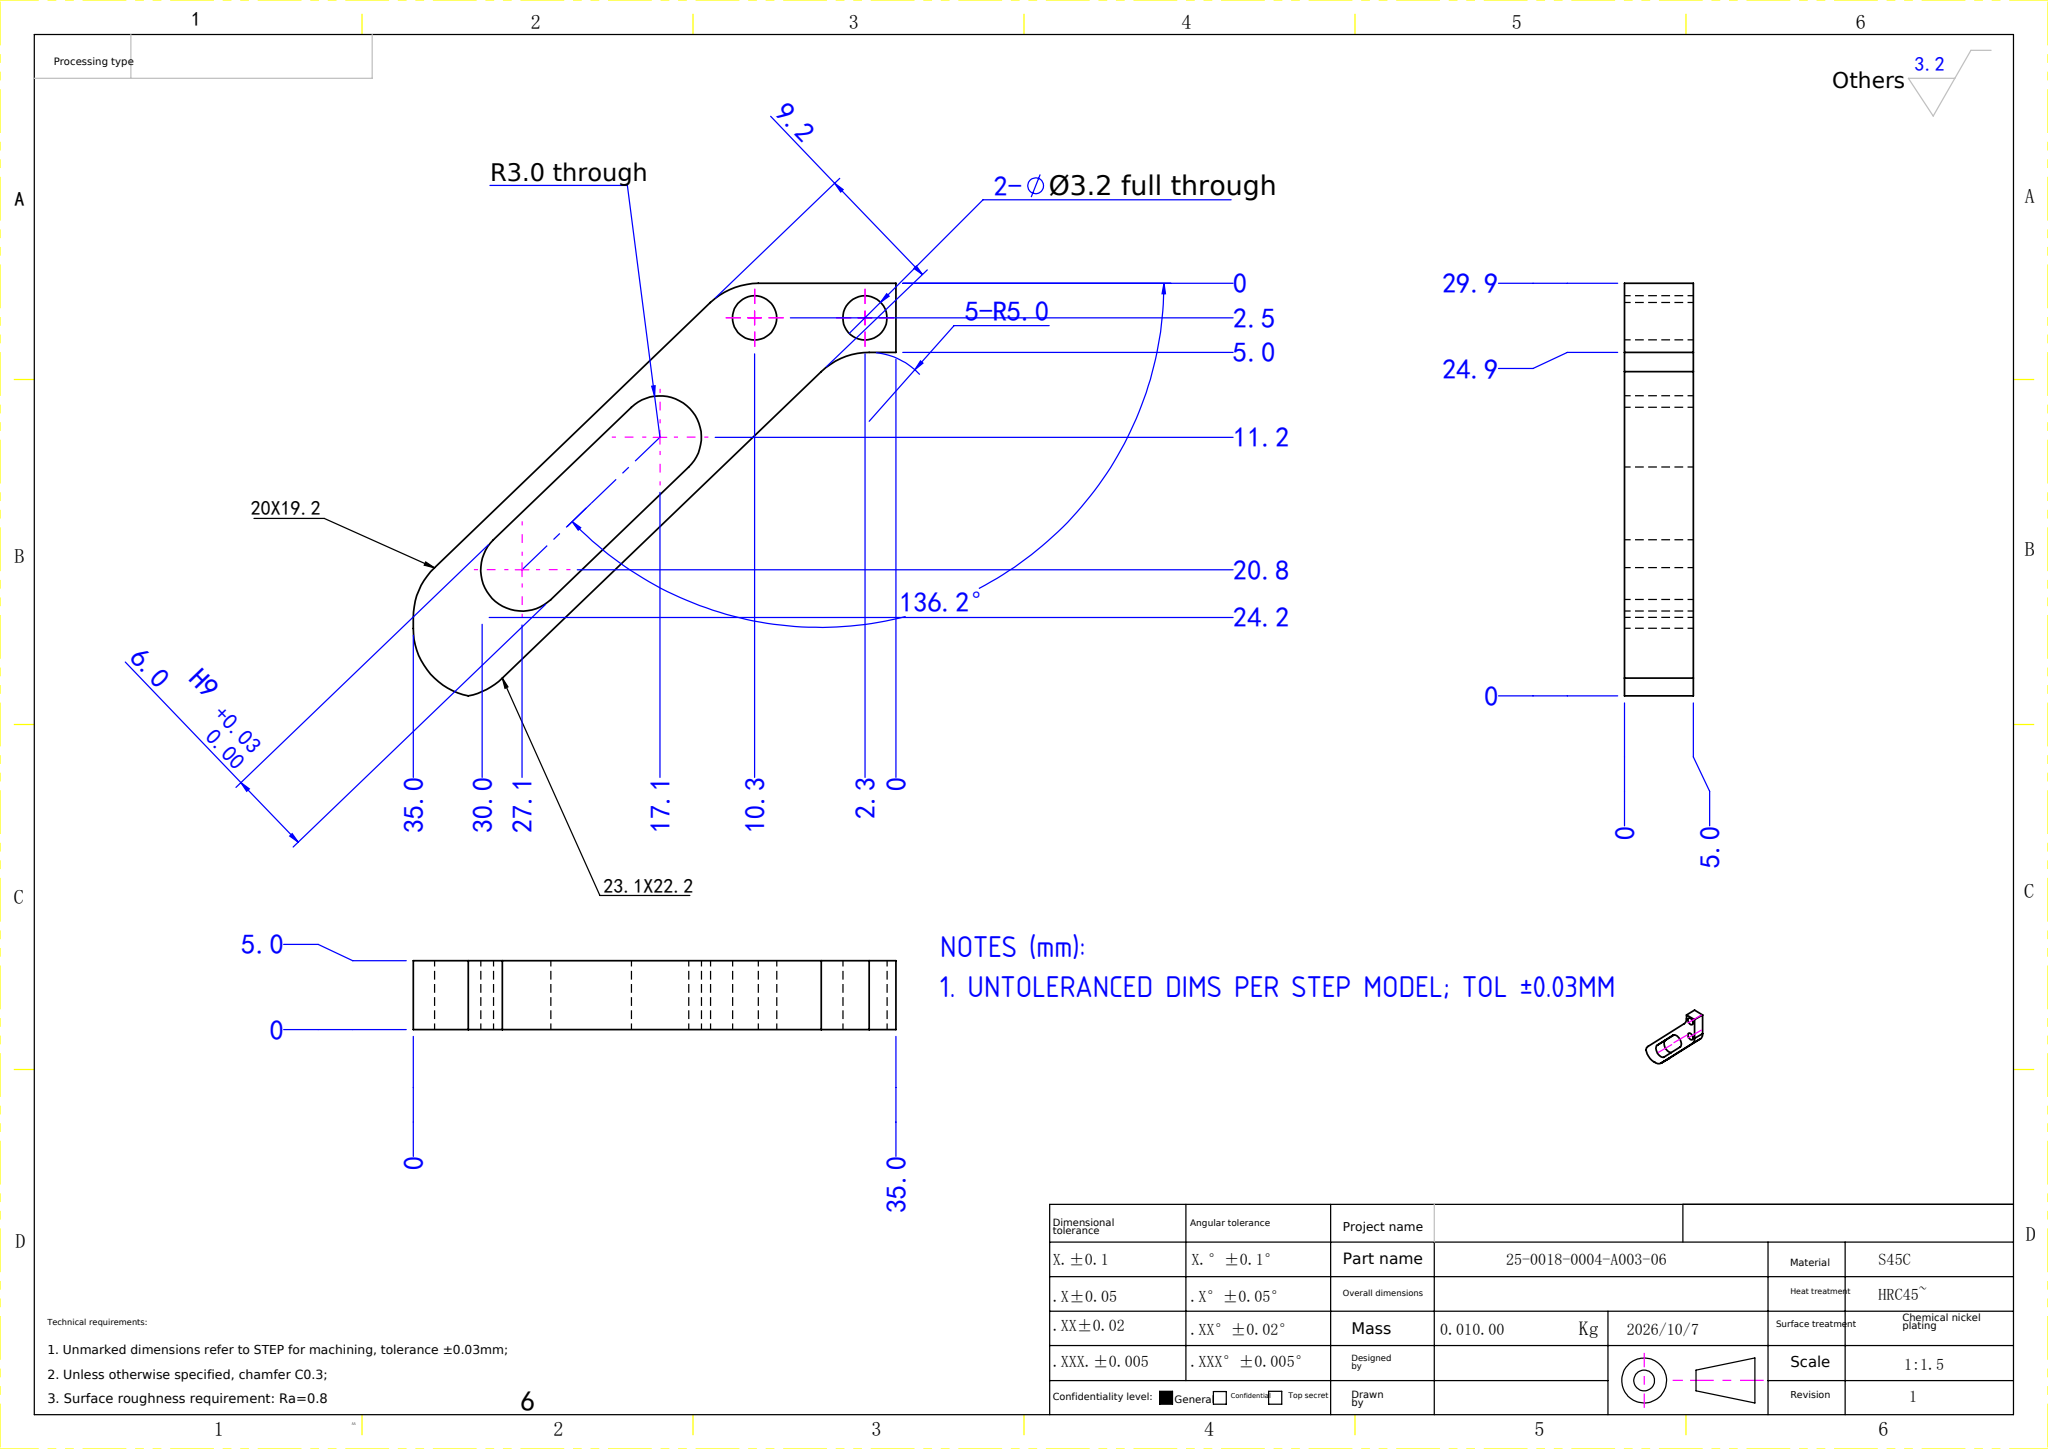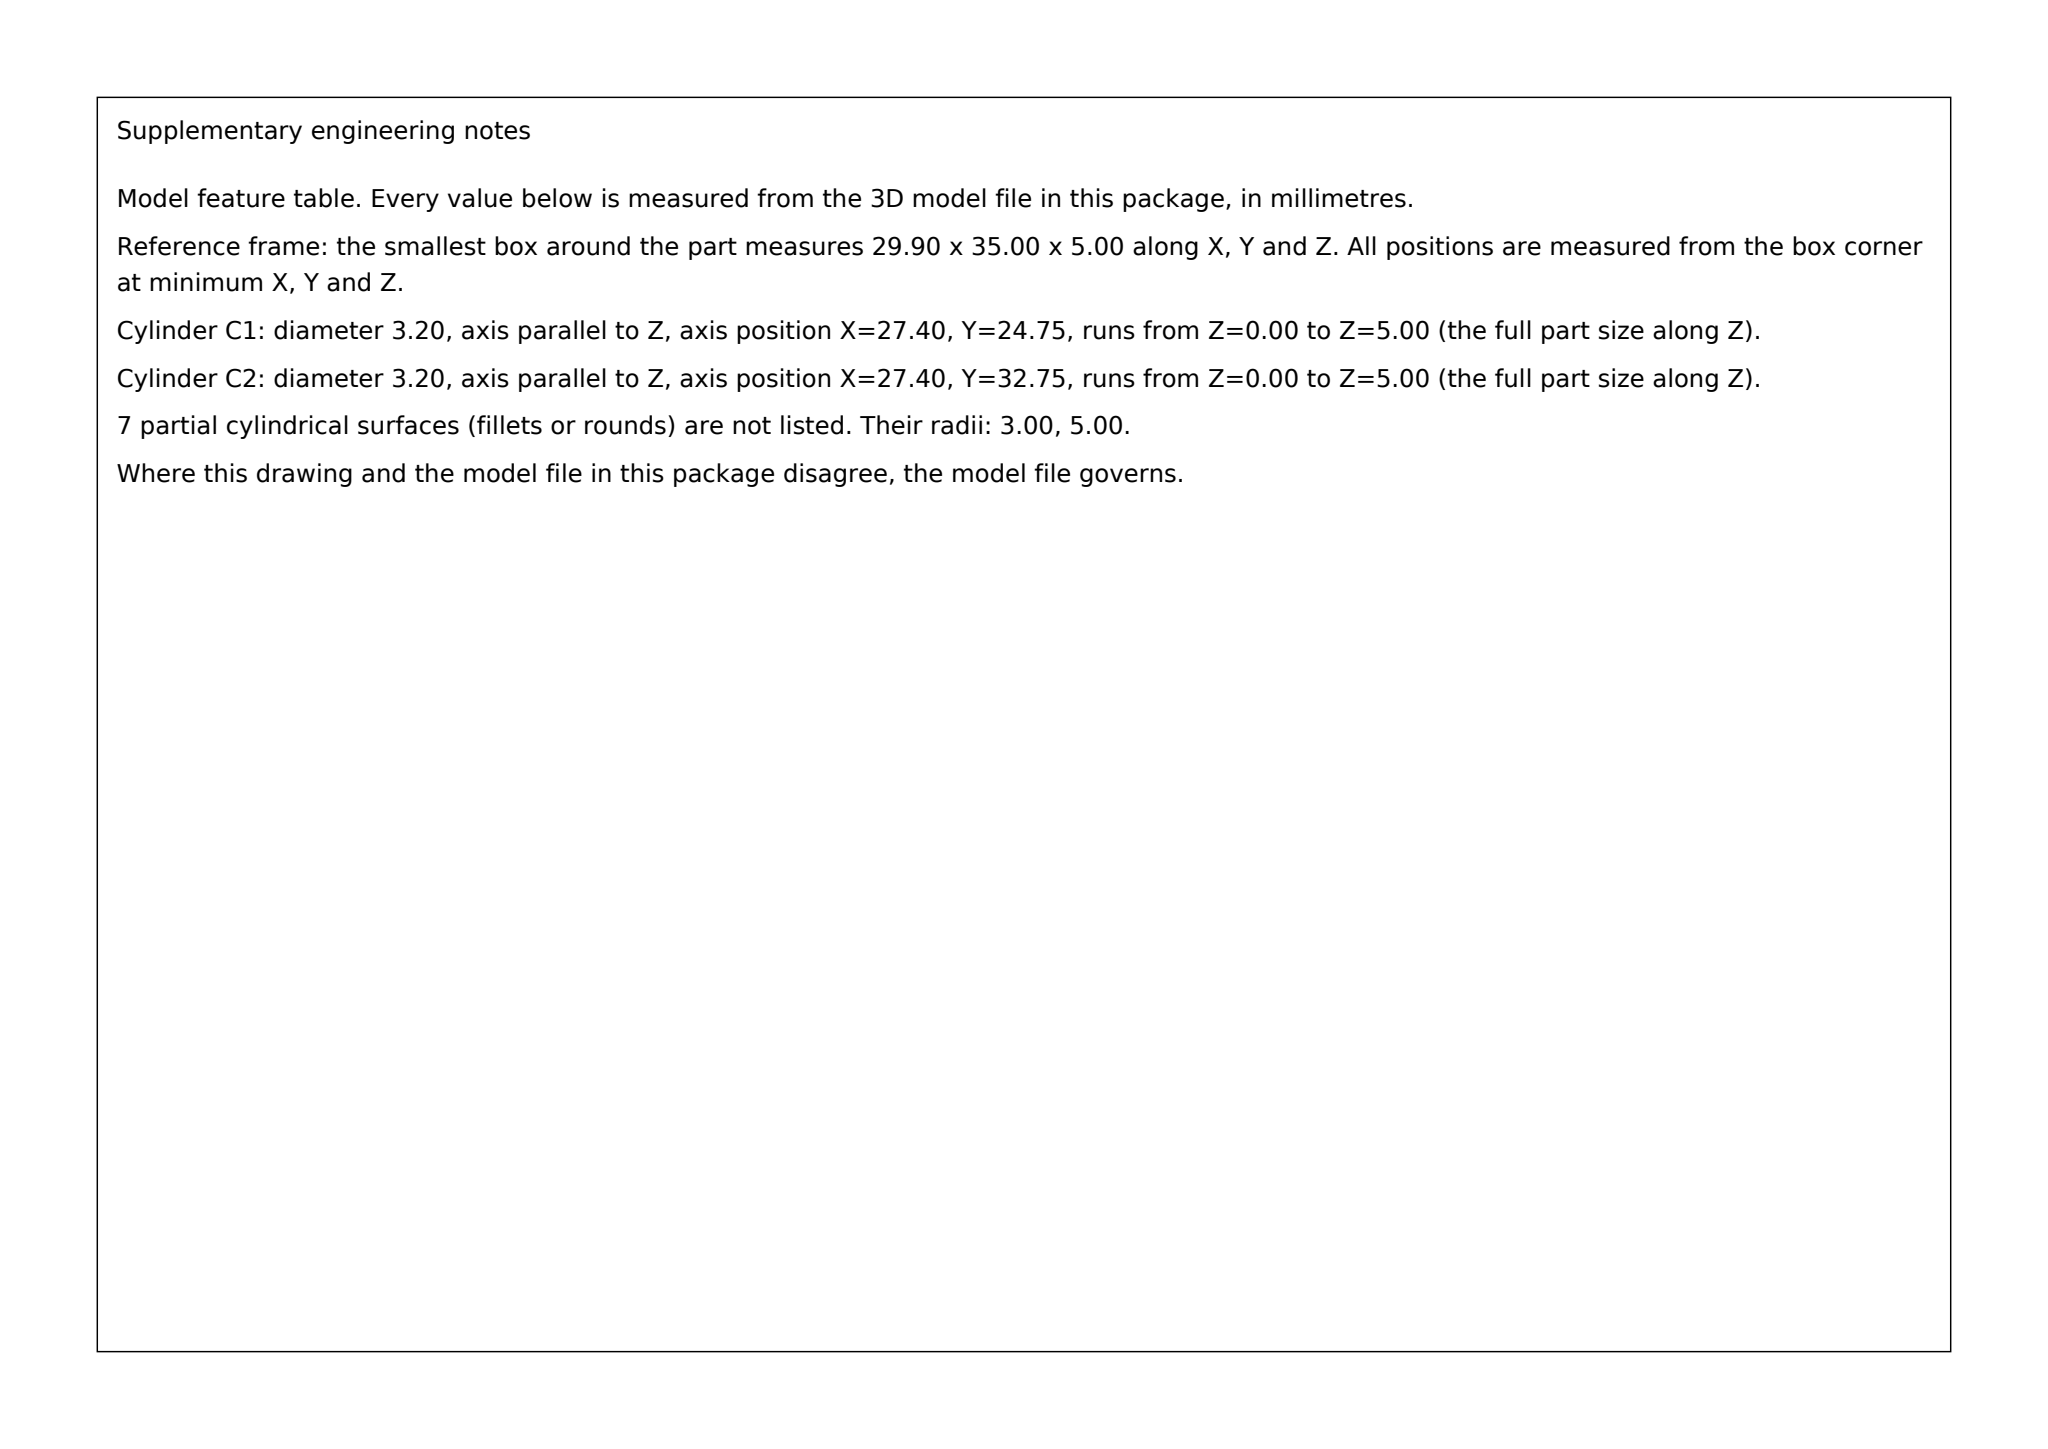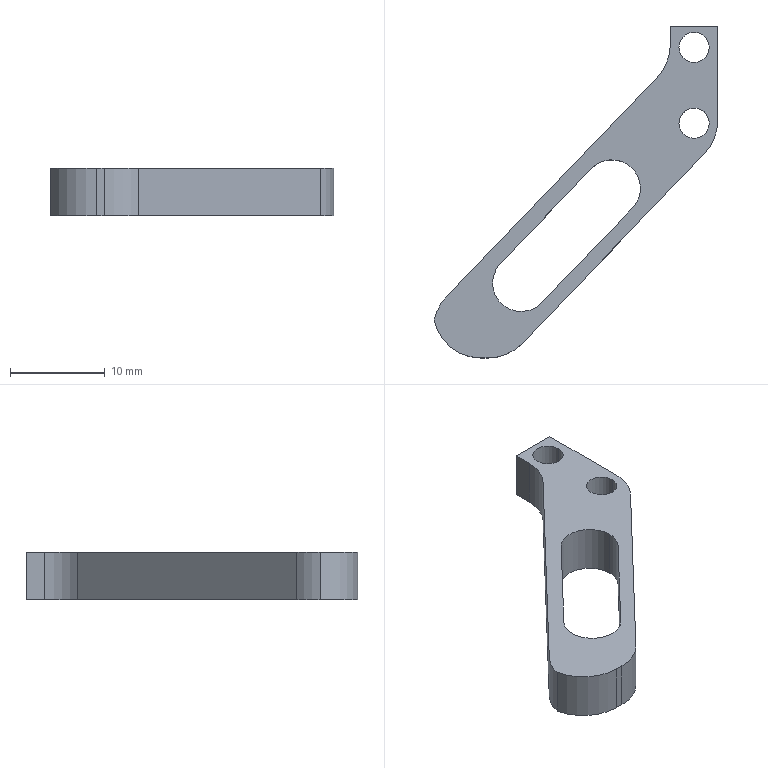Part | SolidWorks | mm | material S45C | 1 solid | 22 faces | box 29.9 x 35 x 5 mm | volume 1188 mm3 | cylinder 12 | plane 10 | commonest cylinder face diameters 10 x5 3.2 x4 6 x3
Drawing notes:
UNTOLERANCED DIMS PER STEP MODEL; TOL ±0.03MM | from the solid: STEP bbox 29.898 x 35.0 x 5.0; all geometry defined in STEP model
STEP:
#1=CARTESIAN_POINT('',(10.9,7.25,-2.5));
#2=VERTEX_POINT('',#1);
#3=CARTESIAN_POINT('',(14.1,7.25,-2.5));
#4=VERTEX_POINT('',#3);
#5=CARTESIAN_POINT('',(12.5,7.25,-2.5));
#6=DIRECTION('',(0.,0.,1.));
#7=DIRECTION('',(1.,0.,0.));
#8=AXIS2_PLACEMENT_3D('',#5,#6,#7);
#9=CIRCLE('',#8,1.6);
#10=EDGE_CURVE('',#2,#4,#9,.T.);
#11=ORIENTED_EDGE('',*,*,#10,.F.);
#12=CARTESIAN_POINT('',(10.9,7.25,2.5));
#13=VERTEX_POINT('',#12);
#14=CARTESIAN_POINT('',(10.9,7.25,2.5));
#15=DIRECTION('',(0.,0.,1.));
#16=VECTOR('',#15,1000.);
#17=LINE('',#14,#16);
#18=EDGE_CURVE('',#2,#13,#17,.T.);
#19=ORIENTED_EDGE('',*,*,#18,.T.);
#20=CARTESIAN_POINT('',(14.1,7.25,2.5));
#21=VERTEX_POINT('',#20);
#22=CARTESIAN_POINT('',(12.5,7.25,2.5));
#23=DIRECTION('',(0.,0.,1.));
#24=DIRECTION('',(1.,0.,0.));
#25=AXIS2_PLACEMENT_3D('',#22,#23,#24);
#26=CIRCLE('',#25,1.6);
#27=EDGE_CURVE('',#13,#21,#26,.T.);
#28=ORIENTED_EDGE('',*,*,#27,.T.);
#29=CARTESIAN_POINT('',(14.1,7.25,2.5));
#30=DIRECTION('',(0.,0.,1.));
#31=VECTOR('',#30,1000.);
#32=LINE('',#29,#31);
#33=EDGE_CURVE('',#4,#21,#32,.T.);
#34=ORIENTED_EDGE('',*,*,#33,.F.);
#35=EDGE_LOOP('',(#11,#19,#28,#34));
#36=FACE_OUTER_BOUND('',#35,.T.);
#37=CARTESIAN_POINT('',(12.5,7.25,2.5));
#38=DIRECTION('',(0.,0.,1.));
#39=DIRECTION('',(1.,0.,0.));
#40=AXIS2_PLACEMENT_3D('',#37,#38,#39);
#41=CYLINDRICAL_SURFACE('',#40,1.6);
#42=ADVANCED_FACE('',(#36),#41,.F.);
#43=CARTESIAN_POINT('',(10.9,15.25,-2.5));
#44=VERTEX_POINT('',#43);
#45=CARTESIAN_POINT('',(14.1,15.25,-2.5));
#46=VERTEX_POINT('',#45);
#47=CARTESIAN_POINT('',(12.5,15.25,-2.5));
#48=DIRECTION('',(0.,0.,1.));
#49=DIRECTION('',(1.,0.,0.));
#50=AXIS2_PLACEMENT_3D('',#47,#48,#49);
#51=CIRCLE('',#50,1.6);
#52=EDGE_CURVE('',#44,#46,#51,.T.);
#53=ORIENTED_EDGE('',*,*,#52,.F.);
#54=CARTESIAN_POINT('',(10.9,15.25,2.5));
#55=VERTEX_POINT('',#54);
#56=CARTESIAN_POINT('',(10.9,15.25,2.5));
#57=DIRECTION('',(0.,0.,1.));
#58=VECTOR('',#57,1000.);
#59=LINE('',#56,#58);
#60=EDGE_CURVE('',#44,#55,#59,.T.);
#61=ORIENTED_EDGE('',*,*,#60,.T.);
#62=CARTESIAN_POINT('',(14.1,15.25,2.5));
#63=VERTEX_POINT('',#62);
#64=CARTESIAN_POINT('',(12.5,15.25,2.5));
#65=DIRECTION('',(0.,0.,1.));
#66=DIRECTION('',(1.,0.,0.));
#67=AXIS2_PLACEMENT_3D('',#64,#65,#66);
#68=CIRCLE('',#67,1.6);
#69=EDGE_CURVE('',#55,#63,#68,.T.);
#70=ORIENTED_EDGE('',*,*,#69,.T.);
#71=CARTESIAN_POINT('',(14.1,15.25,2.5));
#72=DIRECTION('',(0.,0.,1.));
#73=VECTOR('',#72,1000.);
#74=LINE('',#71,#73);
#75=EDGE_CURVE('',#46,#63,#74,.T.);
#76=ORIENTED_EDGE('',*,*,#75,.F.);
#77=EDGE_LOOP('',(#53,#61,#70,#76));
#78=FACE_OUTER_BOUND('',#77,.T.);
#79=CARTESIAN_POINT('',(12.5,15.25,2.5));
#80=DIRECTION('',(0.,0.,1.));
#81=DIRECTION('',(1.,0.,0.));
#82=AXIS2_PLACEMENT_3D('',#79,#80,#81);
#83=CYLINDRICAL_SURFACE('',#82,1.6);
#84=ADVANCED_FACE('',(#78),#83,.F.);
#85=CARTESIAN_POINT('',(6.85,0.39,-2.5));
#86=VERTEX_POINT('',#85);
#87=CARTESIAN_POINT('',(1.686,2.468,-2.5));
#88=VERTEX_POINT('',#87);
#89=CARTESIAN_POINT('',(3.85,0.39,-2.5));
#90=DIRECTION('',(0.,0.,1.));
#91=DIRECTION('',(1.,0.,0.));
#92=AXIS2_PLACEMENT_3D('',#89,#90,#91);
#93=CIRCLE('',#92,3.);
#94=EDGE_CURVE('',#86,#88,#93,.T.);
#95=ORIENTED_EDGE('',*,*,#94,.F.);
#96=CARTESIAN_POINT('',(6.85,0.39,2.5));
#97=VERTEX_POINT('',#96);
#98=CARTESIAN_POINT('',(6.85,0.39,-2.5));
#99=DIRECTION('',(0.,0.,1.));
#100=VECTOR('',#99,1000.);
#101=LINE('',#98,#100);
#102=EDGE_CURVE('',#86,#97,#101,.T.);
#103=ORIENTED_EDGE('',*,*,#102,.T.);
#104=CARTESIAN_POINT('',(1.686,2.468,2.5));
#105=VERTEX_POINT('',#104);
#106=CARTESIAN_POINT('',(3.85,0.39,2.5));
#107=DIRECTION('',(0.,0.,1.));
#108=DIRECTION('',(1.,0.,0.));
#109=AXIS2_PLACEMENT_3D('',#106,#107,#108);
#110=CIRCLE('',#109,3.);
#111=EDGE_CURVE('',#97,#105,#110,.T.);
#112=ORIENTED_EDGE('',*,*,#111,.T.);
#113=CARTESIAN_POINT('',(1.686,2.468,-7.5));
#114=DIRECTION('',(0.,0.,1.));
#115=VECTOR('',#114,1000.);
#116=LINE('',#113,#115);
#117=EDGE_CURVE('',#88,#105,#116,.T.);
#118=ORIENTED_EDGE('',*,*,#117,.F.);
#119=EDGE_LOOP('',(#95,#103,#112,#118));
#120=FACE_OUTER_BOUND('',#119,.T.);
#121=CARTESIAN_POINT('',(3.85,0.39,-2.5));
#122=DIRECTION('',(0.,0.,1.));
#123=DIRECTION('',(1.,0.,0.));
#124=AXIS2_PLACEMENT_3D('',#121,#122,#123);
#125=CYLINDRICAL_SURFACE('',#124,3.);
#126=ADVANCED_FACE('',(#120),#125,.F.);
#127=CARTESIAN_POINT('',(12.5,7.25,2.5));
#128=DIRECTION('',(0.,0.,1.));
#129=DIRECTION('',(1.,0.,0.));
#130=AXIS2_PLACEMENT_3D('',#127,#128,#129);
#131=CIRCLE('',#130,1.6);
#132=EDGE_CURVE('',#21,#13,#131,.T.);
#133=ORIENTED_EDGE('',*,*,#132,.F.);
#134=ORIENTED_EDGE('',*,*,#27,.F.);
#135=EDGE_LOOP('',(#133,#134));
#136=FACE_BOUND('',#135,.T.);
#137=CARTESIAN_POINT('',(6.014,-1.688,2.5));
#138=VERTEX_POINT('',#137);
#139=CARTESIAN_POINT('',(3.85,0.39,2.5));
#140=DIRECTION('',(0.,0.,1.));
#141=DIRECTION('',(1.,0.,0.));
#142=AXIS2_PLACEMENT_3D('',#139,#140,#141);
#143=CIRCLE('',#142,3.);
#144=EDGE_CURVE('',#138,#97,#143,.T.);
#145=ORIENTED_EDGE('',*,*,#144,.F.);
#146=CARTESIAN_POINT('',(-3.586,-11.688,2.5));
#147=VERTEX_POINT('',#146);
#148=CARTESIAN_POINT('',(6.014,-1.688,2.5));
#149=DIRECTION('',(0.6925,0.7214,0.));
#150=VECTOR('',#149,1000.);
#151=LINE('',#148,#150);
#152=EDGE_CURVE('',#147,#138,#151,.T.);
#153=ORIENTED_EDGE('',*,*,#152,.F.);
#154=CARTESIAN_POINT('',(-7.914,-7.532,2.5));
#155=VERTEX_POINT('',#154);
#156=CARTESIAN_POINT('',(-5.75,-9.61,2.5));
#157=DIRECTION('',(0.,0.,1.));
#158=DIRECTION('',(1.,0.,0.));
#159=AXIS2_PLACEMENT_3D('',#156,#157,#158);
#160=CIRCLE('',#159,3.);
#161=EDGE_CURVE('',#155,#147,#160,.T.);
#162=ORIENTED_EDGE('',*,*,#161,.F.);
#163=CARTESIAN_POINT('',(1.686,2.468,2.5));
#164=DIRECTION('',(-0.6925,-0.7214,0.));
#165=VECTOR('',#164,1000.);
#166=LINE('',#163,#165);
#167=EDGE_CURVE('',#105,#155,#166,.T.);
#168=ORIENTED_EDGE('',*,*,#167,.F.);
#169=ORIENTED_EDGE('',*,*,#111,.F.);
#170=EDGE_LOOP('',(#145,#153,#162,#168,#169));
#171=FACE_BOUND('',#170,.T.);
#172=CARTESIAN_POINT('',(-13.607,-11.049,2.5));
#173=VERTEX_POINT('',#172);
#174=CARTESIAN_POINT('',(-14.898,-13.506,2.5));
#175=VERTEX_POINT('',#174);
#176=CARTESIAN_POINT('',(-10.,-14.512,2.5));
#177=DIRECTION('',(0.,0.,1.));
#178=DIRECTION('',(-1.,0.,0.));
#179=AXIS2_PLACEMENT_3D('',#176,#177,#178);
#180=CIRCLE('',#179,5.);
#181=EDGE_CURVE('',#173,#175,#180,.T.);
#182=ORIENTED_EDGE('',*,*,#181,.T.);
#183=CARTESIAN_POINT('',(-10.,-17.5,2.5));
#184=VERTEX_POINT('',#183);
#185=CARTESIAN_POINT('',(-10.,-12.5,2.5));
#186=DIRECTION('',(0.,0.,1.));
#187=DIRECTION('',(-1.,0.,0.));
#188=AXIS2_PLACEMENT_3D('',#185,#186,#187);
#189=CIRCLE('',#188,5.);
#190=EDGE_CURVE('',#175,#184,#189,.T.);
#191=ORIENTED_EDGE('',*,*,#190,.T.);
#192=CARTESIAN_POINT('',(-9.211,-17.5,2.5));
#193=VERTEX_POINT('',#192);
#194=CARTESIAN_POINT('',(-15.,-17.5,2.5));
#195=DIRECTION('',(1.,0.,0.));
#196=VECTOR('',#195,1000.);
#197=LINE('',#194,#196);
#198=EDGE_CURVE('',#184,#193,#197,.T.);
#199=ORIENTED_EDGE('',*,*,#198,.T.);
#200=CARTESIAN_POINT('',(-5.604,-15.963,2.5));
#201=VERTEX_POINT('',#200);
#202=CARTESIAN_POINT('',(-9.211,-12.5,2.5));
#203=DIRECTION('',(0.,0.,1.));
#204=DIRECTION('',(-1.,0.,0.));
#205=AXIS2_PLACEMENT_3D('',#202,#203,#204);
#206=CIRCLE('',#205,5.);
#207=EDGE_CURVE('',#193,#201,#206,.T.);
#208=ORIENTED_EDGE('',*,*,#207,.T.);
#209=CARTESIAN_POINT('',(13.607,4.049,2.5));
#210=VERTEX_POINT('',#209);
#211=CARTESIAN_POINT('',(15.,5.5,2.5));
#212=DIRECTION('',(-0.6925,-0.7214,0.));
#213=VECTOR('',#212,1000.);
#214=LINE('',#211,#213);
#215=EDGE_CURVE('',#210,#201,#214,.T.);
#216=ORIENTED_EDGE('',*,*,#215,.F.);
#217=CARTESIAN_POINT('',(15.,7.512,2.5));
#218=VERTEX_POINT('',#217);
#219=CARTESIAN_POINT('',(10.,7.512,2.5));
#220=DIRECTION('',(0.,0.,1.));
#221=DIRECTION('',(-1.,0.,0.));
#222=AXIS2_PLACEMENT_3D('',#219,#220,#221);
#223=CIRCLE('',#222,5.);
#224=EDGE_CURVE('',#210,#218,#223,.T.);
#225=ORIENTED_EDGE('',*,*,#224,.T.);
#226=CARTESIAN_POINT('',(15.,17.5,2.5));
#227=VERTEX_POINT('',#226);
#228=CARTESIAN_POINT('',(15.,17.5,2.5));
#229=DIRECTION('',(0.,-1.,0.));
#230=VECTOR('',#229,1000.);
#231=LINE('',#228,#230);
#232=EDGE_CURVE('',#227,#218,#231,.T.);
#233=ORIENTED_EDGE('',*,*,#232,.F.);
#234=CARTESIAN_POINT('',(10.,17.5,2.5));
#235=VERTEX_POINT('',#234);
#236=CARTESIAN_POINT('',(-15.,17.5,2.5));
#237=DIRECTION('',(1.,0.,0.));
#238=VECTOR('',#237,1000.);
#239=LINE('',#236,#238);
#240=EDGE_CURVE('',#235,#227,#239,.T.);
#241=ORIENTED_EDGE('',*,*,#240,.F.);
#242=CARTESIAN_POINT('',(10.,15.553,2.5));
#243=VERTEX_POINT('',#242);
#244=CARTESIAN_POINT('',(10.,17.5,2.5));
#245=DIRECTION('',(0.,1.,0.));
#246=VECTOR('',#245,1000.);
#247=LINE('',#244,#246);
#248=EDGE_CURVE('',#243,#235,#247,.T.);
#249=ORIENTED_EDGE('',*,*,#248,.F.);
#250=CARTESIAN_POINT('',(8.607,12.091,2.5));
#251=VERTEX_POINT('',#250);
#252=CARTESIAN_POINT('',(5.,15.553,2.5));
#253=DIRECTION('',(0.,0.,-1.));
#254=DIRECTION('',(-1.,0.,0.));
#255=AXIS2_PLACEMENT_3D('',#252,#253,#254);
#256=CIRCLE('',#255,5.);
#257=EDGE_CURVE('',#243,#251,#256,.T.);
#258=ORIENTED_EDGE('',*,*,#257,.T.);
#259=CARTESIAN_POINT('',(10.,13.542,2.5));
#260=DIRECTION('',(0.6925,0.7214,0.));
#261=VECTOR('',#260,1000.);
#262=LINE('',#259,#261);
#263=EDGE_CURVE('',#173,#251,#262,.T.);
#264=ORIENTED_EDGE('',*,*,#263,.F.);
#265=EDGE_LOOP('',(#182,#191,#199,#208,#216,#225,#233,#241,#249,#258,#264));
#266=FACE_OUTER_BOUND('',#265,.T.);
#267=CARTESIAN_POINT('',(12.5,15.25,2.5));
#268=DIRECTION('',(0.,0.,1.));
#269=DIRECTION('',(1.,0.,0.));
#270=AXIS2_PLACEMENT_3D('',#267,#268,#269);
#271=CIRCLE('',#270,1.6);
#272=EDGE_CURVE('',#63,#55,#271,.T.);
#273=ORIENTED_EDGE('',*,*,#272,.F.);
#274=ORIENTED_EDGE('',*,*,#69,.F.);
#275=EDGE_LOOP('',(#273,#274));
#276=FACE_BOUND('',#275,.T.);
#277=CARTESIAN_POINT('',(-15.,17.5,2.5));
#278=DIRECTION('',(0.,0.,-1.));
#279=DIRECTION('',(-1.,0.,0.));
#280=AXIS2_PLACEMENT_3D('',#277,#278,#279);
#281=PLANE('',#280);
#282=ADVANCED_FACE('',(#136,#171,#266,#276),#281,.F.);
#283=ORIENTED_EDGE('',*,*,#102,.F.);
#284=CARTESIAN_POINT('',(6.014,-1.688,-2.5));
#285=VERTEX_POINT('',#284);
#286=CARTESIAN_POINT('',(3.85,0.39,-2.5));
#287=DIRECTION('',(0.,0.,1.));
#288=DIRECTION('',(1.,0.,0.));
#289=AXIS2_PLACEMENT_3D('',#286,#287,#288);
#290=CIRCLE('',#289,3.);
#291=EDGE_CURVE('',#285,#86,#290,.T.);
#292=ORIENTED_EDGE('',*,*,#291,.F.);
#293=CARTESIAN_POINT('',(6.014,-1.688,-7.5));
#294=DIRECTION('',(0.,0.,1.));
#295=VECTOR('',#294,1000.);
#296=LINE('',#293,#295);
#297=EDGE_CURVE('',#285,#138,#296,.T.);
#298=ORIENTED_EDGE('',*,*,#297,.T.);
#299=ORIENTED_EDGE('',*,*,#144,.T.);
#300=EDGE_LOOP('',(#283,#292,#298,#299));
#301=FACE_OUTER_BOUND('',#300,.T.);
#302=CARTESIAN_POINT('',(3.85,0.39,-2.5));
#303=DIRECTION('',(0.,0.,1.));
#304=DIRECTION('',(1.,0.,0.));
#305=AXIS2_PLACEMENT_3D('',#302,#303,#304);
#306=CYLINDRICAL_SURFACE('',#305,3.);
#307=ADVANCED_FACE('',(#301),#306,.F.);
#308=ORIENTED_EDGE('',*,*,#232,.T.);
#309=CARTESIAN_POINT('',(15.,7.512,-2.5));
#310=VERTEX_POINT('',#309);
#311=CARTESIAN_POINT('',(15.,7.512,-2.5));
#312=DIRECTION('',(0.,0.,-1.));
#313=VECTOR('',#312,1000.);
#314=LINE('',#311,#313);
#315=EDGE_CURVE('',#218,#310,#314,.T.);
#316=ORIENTED_EDGE('',*,*,#315,.T.);
#317=CARTESIAN_POINT('',(15.,17.5,-2.5));
#318=VERTEX_POINT('',#317);
#319=CARTESIAN_POINT('',(15.,17.5,-2.5));
#320=DIRECTION('',(0.,-1.,0.));
#321=VECTOR('',#320,1000.);
#322=LINE('',#319,#321);
#323=EDGE_CURVE('',#318,#310,#322,.T.);
#324=ORIENTED_EDGE('',*,*,#323,.F.);
#325=CARTESIAN_POINT('',(15.,17.5,-2.5));
#326=DIRECTION('',(0.,0.,-1.));
#327=VECTOR('',#326,1000.);
#328=LINE('',#325,#327);
#329=EDGE_CURVE('',#227,#318,#328,.T.);
#330=ORIENTED_EDGE('',*,*,#329,.F.);
#331=EDGE_LOOP('',(#308,#316,#324,#330));
#332=FACE_OUTER_BOUND('',#331,.T.);
#333=CARTESIAN_POINT('',(15.,17.5,-2.5));
#334=DIRECTION('',(-1.,0.,0.));
#335=DIRECTION('',(0.,0.,1.));
#336=AXIS2_PLACEMENT_3D('',#333,#334,#335);
#337=PLANE('',#336);
#338=ADVANCED_FACE('',(#332),#337,.F.);
#339=CARTESIAN_POINT('',(12.5,7.25,-2.5));
#340=DIRECTION('',(0.,0.,1.));
#341=DIRECTION('',(1.,0.,0.));
#342=AXIS2_PLACEMENT_3D('',#339,#340,#341);
#343=CIRCLE('',#342,1.6);
#344=EDGE_CURVE('',#4,#2,#343,.T.);
#345=ORIENTED_EDGE('',*,*,#344,.T.);
#346=ORIENTED_EDGE('',*,*,#10,.T.);
#347=EDGE_LOOP('',(#345,#346));
#348=FACE_BOUND('',#347,.T.);
#349=CARTESIAN_POINT('',(12.5,15.25,-2.5));
#350=DIRECTION('',(0.,0.,1.));
#351=DIRECTION('',(1.,0.,0.));
#352=AXIS2_PLACEMENT_3D('',#349,#350,#351);
#353=CIRCLE('',#352,1.6);
#354=EDGE_CURVE('',#46,#44,#353,.T.);
#355=ORIENTED_EDGE('',*,*,#354,.T.);
#356=ORIENTED_EDGE('',*,*,#52,.T.);
#357=EDGE_LOOP('',(#355,#356));
#358=FACE_BOUND('',#357,.T.);
#359=CARTESIAN_POINT('',(-7.914,-7.532,-2.5));
#360=VERTEX_POINT('',#359);
#361=CARTESIAN_POINT('',(-3.586,-11.688,-2.5));
#362=VERTEX_POINT('',#361);
#363=CARTESIAN_POINT('',(-5.75,-9.61,-2.5));
#364=DIRECTION('',(0.,0.,1.));
#365=DIRECTION('',(1.,0.,0.));
#366=AXIS2_PLACEMENT_3D('',#363,#364,#365);
#367=CIRCLE('',#366,3.);
#368=EDGE_CURVE('',#360,#362,#367,.T.);
#369=ORIENTED_EDGE('',*,*,#368,.T.);
#370=CARTESIAN_POINT('',(5.522,-2.201,-2.5));
#371=DIRECTION('',(0.6925,0.7214,0.));
#372=VECTOR('',#371,1000.);
#373=LINE('',#370,#372);
#374=EDGE_CURVE('',#362,#285,#373,.T.);
#375=ORIENTED_EDGE('',*,*,#374,.T.);
#376=ORIENTED_EDGE('',*,*,#291,.T.);
#377=ORIENTED_EDGE('',*,*,#94,.T.);
#378=CARTESIAN_POINT('',(1.193,1.954,-2.5));
#379=DIRECTION('',(-0.6925,-0.7214,0.));
#380=VECTOR('',#379,1000.);
#381=LINE('',#378,#380);
#382=EDGE_CURVE('',#88,#360,#381,.T.);
#383=ORIENTED_EDGE('',*,*,#382,.T.);
#384=EDGE_LOOP('',(#369,#375,#376,#377,#383));
#385=FACE_BOUND('',#384,.T.);
#386=CARTESIAN_POINT('',(-9.211,-17.5,-2.5));
#387=VERTEX_POINT('',#386);
#388=CARTESIAN_POINT('',(-10.,-17.5,-2.5));
#389=VERTEX_POINT('',#388);
#390=CARTESIAN_POINT('',(-15.,-17.5,-2.5));
#391=DIRECTION('',(-1.,0.,0.));
#392=VECTOR('',#391,1000.);
#393=LINE('',#390,#392);
#394=EDGE_CURVE('',#387,#389,#393,.T.);
#395=ORIENTED_EDGE('',*,*,#394,.T.);
#396=CARTESIAN_POINT('',(-14.898,-13.506,-2.5));
#397=VERTEX_POINT('',#396);
#398=CARTESIAN_POINT('',(-10.,-12.5,-2.5));
#399=DIRECTION('',(0.,0.,-1.));
#400=DIRECTION('',(1.,0.,0.));
#401=AXIS2_PLACEMENT_3D('',#398,#399,#400);
#402=CIRCLE('',#401,5.);
#403=EDGE_CURVE('',#389,#397,#402,.T.);
#404=ORIENTED_EDGE('',*,*,#403,.T.);
#405=CARTESIAN_POINT('',(-13.607,-11.049,-2.5));
#406=VERTEX_POINT('',#405);
#407=CARTESIAN_POINT('',(-10.,-14.512,-2.5));
#408=DIRECTION('',(0.,0.,-1.));
#409=DIRECTION('',(1.,0.,0.));
#410=AXIS2_PLACEMENT_3D('',#407,#408,#409);
#411=CIRCLE('',#410,5.);
#412=EDGE_CURVE('',#397,#406,#411,.T.);
#413=ORIENTED_EDGE('',*,*,#412,.T.);
#414=CARTESIAN_POINT('',(8.607,12.091,-2.5));
#415=VERTEX_POINT('',#414);
#416=CARTESIAN_POINT('',(10.,13.542,-2.5));
#417=DIRECTION('',(0.6925,0.7214,0.));
#418=VECTOR('',#417,1000.);
#419=LINE('',#416,#418);
#420=EDGE_CURVE('',#406,#415,#419,.T.);
#421=ORIENTED_EDGE('',*,*,#420,.T.);
#422=CARTESIAN_POINT('',(10.,15.553,-2.5));
#423=VERTEX_POINT('',#422);
#424=CARTESIAN_POINT('',(5.,15.553,-2.5));
#425=DIRECTION('',(0.,0.,1.));
#426=DIRECTION('',(1.,0.,0.));
#427=AXIS2_PLACEMENT_3D('',#424,#425,#426);
#428=CIRCLE('',#427,5.);
#429=EDGE_CURVE('',#415,#423,#428,.T.);
#430=ORIENTED_EDGE('',*,*,#429,.T.);
#431=CARTESIAN_POINT('',(10.,17.5,-2.5));
#432=VERTEX_POINT('',#431);
#433=CARTESIAN_POINT('',(10.,17.5,-2.5));
#434=DIRECTION('',(0.,1.,0.));
#435=VECTOR('',#434,1000.);
#436=LINE('',#433,#435);
#437=EDGE_CURVE('',#423,#432,#436,.T.);
#438=ORIENTED_EDGE('',*,*,#437,.T.);
#439=CARTESIAN_POINT('',(-15.,17.5,-2.5));
#440=DIRECTION('',(-1.,0.,0.));
#441=VECTOR('',#440,1000.);
#442=LINE('',#439,#441);
#443=EDGE_CURVE('',#318,#432,#442,.T.);
#444=ORIENTED_EDGE('',*,*,#443,.F.);
#445=ORIENTED_EDGE('',*,*,#323,.T.);
#446=CARTESIAN_POINT('',(13.607,4.049,-2.5));
#447=VERTEX_POINT('',#446);
#448=CARTESIAN_POINT('',(10.,7.512,-2.5));
#449=DIRECTION('',(0.,0.,-1.));
#450=DIRECTION('',(1.,0.,0.));
#451=AXIS2_PLACEMENT_3D('',#448,#449,#450);
#452=CIRCLE('',#451,5.);
#453=EDGE_CURVE('',#310,#447,#452,.T.);
#454=ORIENTED_EDGE('',*,*,#453,.T.);
#455=CARTESIAN_POINT('',(-5.604,-15.963,-2.5));
#456=VERTEX_POINT('',#455);
#457=CARTESIAN_POINT('',(15.,5.5,-2.5));
#458=DIRECTION('',(-0.6925,-0.7214,0.));
#459=VECTOR('',#458,1000.);
#460=LINE('',#457,#459);
#461=EDGE_CURVE('',#447,#456,#460,.T.);
#462=ORIENTED_EDGE('',*,*,#461,.T.);
#463=CARTESIAN_POINT('',(-9.211,-12.5,-2.5));
#464=DIRECTION('',(0.,0.,-1.));
#465=DIRECTION('',(1.,0.,0.));
#466=AXIS2_PLACEMENT_3D('',#463,#464,#465);
#467=CIRCLE('',#466,5.);
#468=EDGE_CURVE('',#456,#387,#467,.T.);
#469=ORIENTED_EDGE('',*,*,#468,.T.);
#470=EDGE_LOOP('',(#395,#404,#413,#421,#430,#438,#444,#445,#454,#462,#469));
#471=FACE_OUTER_BOUND('',#470,.T.);
#472=CARTESIAN_POINT('',(-15.,17.5,-2.5));
#473=DIRECTION('',(0.,0.,1.));
#474=DIRECTION('',(1.,0.,0.));
#475=AXIS2_PLACEMENT_3D('',#472,#473,#474);
#476=PLANE('',#475);
#477=ADVANCED_FACE('',(#348,#358,#385,#471),#476,.F.);
#478=CARTESIAN_POINT('',(10.,17.5,-2.5));
#479=DIRECTION('',(0.,0.,1.));
#480=VECTOR('',#479,1000.);
#481=LINE('',#478,#480);
#482=EDGE_CURVE('',#432,#235,#481,.T.);
#483=ORIENTED_EDGE('',*,*,#482,.T.);
#484=ORIENTED_EDGE('',*,*,#240,.T.);
#485=ORIENTED_EDGE('',*,*,#329,.T.);
#486=ORIENTED_EDGE('',*,*,#443,.T.);
#487=EDGE_LOOP('',(#483,#484,#485,#486));
#488=FACE_OUTER_BOUND('',#487,.T.);
#489=CARTESIAN_POINT('',(0.,17.5,0.));
#490=DIRECTION('',(0.,1.,0.));
#491=DIRECTION('',(0.,0.,1.));
#492=AXIS2_PLACEMENT_3D('',#489,#490,#491);
#493=PLANE('',#492);
#494=ADVANCED_FACE('',(#488),#493,.T.);
#495=ORIENTED_EDGE('',*,*,#198,.F.);
#496=CARTESIAN_POINT('',(-10.,-17.5,0.));
#497=DIRECTION('',(0.,0.,-1.));
#498=VECTOR('',#497,1000.);
#499=LINE('',#496,#498);
#500=EDGE_CURVE('',#184,#389,#499,.T.);
#501=ORIENTED_EDGE('',*,*,#500,.T.);
#502=ORIENTED_EDGE('',*,*,#394,.F.);
#503=CARTESIAN_POINT('',(-9.211,-17.5,0.));
#504=DIRECTION('',(0.,0.,1.));
#505=VECTOR('',#504,1000.);
#506=LINE('',#503,#505);
#507=EDGE_CURVE('',#387,#193,#506,.T.);
#508=ORIENTED_EDGE('',*,*,#507,.T.);
#509=EDGE_LOOP('',(#495,#501,#502,#508));
#510=FACE_OUTER_BOUND('',#509,.T.);
#511=CARTESIAN_POINT('',(0.,-17.5,0.));
#512=DIRECTION('',(0.,1.,0.));
#513=DIRECTION('',(0.,0.,1.));
#514=AXIS2_PLACEMENT_3D('',#511,#512,#513);
#515=PLANE('',#514);
#516=ADVANCED_FACE('',(#510),#515,.F.);
#517=ORIENTED_EDGE('',*,*,#161,.T.);
#518=CARTESIAN_POINT('',(-3.586,-11.688,-2.5));
#519=DIRECTION('',(0.,0.,-1.));
#520=VECTOR('',#519,1000.);
#521=LINE('',#518,#520);
#522=EDGE_CURVE('',#147,#362,#521,.T.);
#523=ORIENTED_EDGE('',*,*,#522,.T.);
#524=ORIENTED_EDGE('',*,*,#368,.F.);
#525=CARTESIAN_POINT('',(-7.914,-7.532,-2.5));
#526=DIRECTION('',(0.,0.,-1.));
#527=VECTOR('',#526,1000.);
#528=LINE('',#525,#527);
#529=EDGE_CURVE('',#155,#360,#528,.T.);
#530=ORIENTED_EDGE('',*,*,#529,.F.);
#531=EDGE_LOOP('',(#517,#523,#524,#530));
#532=FACE_OUTER_BOUND('',#531,.T.);
#533=CARTESIAN_POINT('',(-5.75,-9.61,-2.5));
#534=DIRECTION('',(0.,0.,1.));
#535=DIRECTION('',(1.,0.,0.));
#536=AXIS2_PLACEMENT_3D('',#533,#534,#535);
#537=CYLINDRICAL_SURFACE('',#536,3.);
#538=ADVANCED_FACE('',(#532),#537,.F.);
#539=ORIENTED_EDGE('',*,*,#117,.T.);
#540=ORIENTED_EDGE('',*,*,#167,.T.);
#541=ORIENTED_EDGE('',*,*,#529,.T.);
#542=ORIENTED_EDGE('',*,*,#382,.F.);
#543=EDGE_LOOP('',(#539,#540,#541,#542));
#544=FACE_OUTER_BOUND('',#543,.T.);
#545=CARTESIAN_POINT('',(1.686,2.468,-7.5));
#546=DIRECTION('',(-0.7214,0.6925,0.));
#547=DIRECTION('',(-0.6925,-0.7214,0.));
#548=AXIS2_PLACEMENT_3D('',#545,#546,#547);
#549=PLANE('',#548);
#550=ADVANCED_FACE('',(#544),#549,.F.);
#551=ORIENTED_EDGE('',*,*,#522,.F.);
#552=ORIENTED_EDGE('',*,*,#152,.T.);
#553=ORIENTED_EDGE('',*,*,#297,.F.);
#554=ORIENTED_EDGE('',*,*,#374,.F.);
#555=EDGE_LOOP('',(#551,#552,#553,#554));
#556=FACE_OUTER_BOUND('',#555,.T.);
#557=CARTESIAN_POINT('',(6.014,-1.688,-7.5));
#558=DIRECTION('',(0.7214,-0.6925,0.));
#559=DIRECTION('',(0.6925,0.7214,0.));
#560=AXIS2_PLACEMENT_3D('',#557,#558,#559);
#561=PLANE('',#560);
#562=ADVANCED_FACE('',(#556),#561,.F.);
#563=ORIENTED_EDGE('',*,*,#437,.F.);
#564=CARTESIAN_POINT('',(10.,15.553,2.5));
#565=DIRECTION('',(0.,0.,1.));
#566=VECTOR('',#565,1000.);
#567=LINE('',#564,#566);
#568=EDGE_CURVE('',#423,#243,#567,.T.);
#569=ORIENTED_EDGE('',*,*,#568,.T.);
#570=ORIENTED_EDGE('',*,*,#248,.T.);
#571=ORIENTED_EDGE('',*,*,#482,.F.);
#572=EDGE_LOOP('',(#563,#569,#570,#571));
#573=FACE_OUTER_BOUND('',#572,.T.);
#574=CARTESIAN_POINT('',(10.,17.5,-2.5));
#575=DIRECTION('',(1.,0.,0.));
#576=DIRECTION('',(0.,0.,-1.));
#577=AXIS2_PLACEMENT_3D('',#574,#575,#576);
#578=PLANE('',#577);
#579=ADVANCED_FACE('',(#573),#578,.F.);
#580=ORIENTED_EDGE('',*,*,#420,.F.);
#581=CARTESIAN_POINT('',(-13.607,-11.049,-2.5));
#582=DIRECTION('',(0.,0.,1.));
#583=VECTOR('',#582,1000.);
#584=LINE('',#581,#583);
#585=EDGE_CURVE('',#406,#173,#584,.T.);
#586=ORIENTED_EDGE('',*,*,#585,.T.);
#587=ORIENTED_EDGE('',*,*,#263,.T.);
#588=CARTESIAN_POINT('',(8.607,12.091,-2.5));
#589=DIRECTION('',(0.,0.,-1.));
#590=VECTOR('',#589,1000.);
#591=LINE('',#588,#590);
#592=EDGE_CURVE('',#251,#415,#591,.T.);
#593=ORIENTED_EDGE('',*,*,#592,.T.);
#594=EDGE_LOOP('',(#580,#586,#587,#593));
#595=FACE_OUTER_BOUND('',#594,.T.);
#596=CARTESIAN_POINT('',(10.,13.542,-2.5));
#597=DIRECTION('',(0.7214,-0.6925,0.));
#598=DIRECTION('',(0.6925,0.7214,0.));
#599=AXIS2_PLACEMENT_3D('',#596,#597,#598);
#600=PLANE('',#599);
#601=ADVANCED_FACE('',(#595),#600,.F.);
#602=ORIENTED_EDGE('',*,*,#215,.T.);
#603=CARTESIAN_POINT('',(-5.604,-15.963,-2.5));
#604=DIRECTION('',(0.,0.,-1.));
#605=VECTOR('',#604,1000.);
#606=LINE('',#603,#605);
#607=EDGE_CURVE('',#201,#456,#606,.T.);
#608=ORIENTED_EDGE('',*,*,#607,.T.);
#609=ORIENTED_EDGE('',*,*,#461,.F.);
#610=CARTESIAN_POINT('',(13.607,4.049,-2.5));
#611=DIRECTION('',(0.,0.,1.));
#612=VECTOR('',#611,1000.);
#613=LINE('',#610,#612);
#614=EDGE_CURVE('',#447,#210,#613,.T.);
#615=ORIENTED_EDGE('',*,*,#614,.T.);
#616=EDGE_LOOP('',(#602,#608,#609,#615));
#617=FACE_OUTER_BOUND('',#616,.T.);
#618=CARTESIAN_POINT('',(15.,5.5,-2.5));
#619=DIRECTION('',(-0.7214,0.6925,0.));
#620=DIRECTION('',(-0.6925,-0.7214,0.));
#621=AXIS2_PLACEMENT_3D('',#618,#619,#620);
#622=PLANE('',#621);
#623=ADVANCED_FACE('',(#617),#622,.F.);
#624=ORIENTED_EDGE('',*,*,#585,.F.);
#625=ORIENTED_EDGE('',*,*,#412,.F.);
#626=CARTESIAN_POINT('',(-14.898,-13.506,-0.));
#627=DIRECTION('',(0.,0.,-1.));
#628=VECTOR('',#627,1000.);
#629=LINE('',#626,#628);
#630=EDGE_CURVE('',#175,#397,#629,.T.);
#631=ORIENTED_EDGE('',*,*,#630,.F.);
#632=ORIENTED_EDGE('',*,*,#181,.F.);
#633=EDGE_LOOP('',(#624,#625,#631,#632));
#634=FACE_OUTER_BOUND('',#633,.T.);
#635=CARTESIAN_POINT('',(-10.,-14.512,-2.5));
#636=DIRECTION('',(0.,0.,1.));
#637=DIRECTION('',(1.,0.,0.));
#638=AXIS2_PLACEMENT_3D('',#635,#636,#637);
#639=CYLINDRICAL_SURFACE('',#638,5.);
#640=ADVANCED_FACE('',(#634),#639,.T.);
#641=ORIENTED_EDGE('',*,*,#403,.F.);
#642=ORIENTED_EDGE('',*,*,#500,.F.);
#643=ORIENTED_EDGE('',*,*,#190,.F.);
#644=ORIENTED_EDGE('',*,*,#630,.T.);
#645=EDGE_LOOP('',(#641,#642,#643,#644));
#646=FACE_OUTER_BOUND('',#645,.T.);
#647=CARTESIAN_POINT('',(-10.,-12.5,-2.5));
#648=DIRECTION('',(0.,0.,1.));
#649=DIRECTION('',(1.,0.,0.));
#650=AXIS2_PLACEMENT_3D('',#647,#648,#649);
#651=CYLINDRICAL_SURFACE('',#650,5.);
#652=ADVANCED_FACE('',(#646),#651,.T.);
#653=ORIENTED_EDGE('',*,*,#468,.F.);
#654=ORIENTED_EDGE('',*,*,#607,.F.);
#655=ORIENTED_EDGE('',*,*,#207,.F.);
#656=ORIENTED_EDGE('',*,*,#507,.F.);
#657=EDGE_LOOP('',(#653,#654,#655,#656));
#658=FACE_OUTER_BOUND('',#657,.T.);
#659=CARTESIAN_POINT('',(-9.211,-12.5,0.));
#660=DIRECTION('',(0.,0.,1.));
#661=DIRECTION('',(1.,0.,0.));
#662=AXIS2_PLACEMENT_3D('',#659,#660,#661);
#663=CYLINDRICAL_SURFACE('',#662,5.);
#664=ADVANCED_FACE('',(#658),#663,.T.);
#665=ORIENTED_EDGE('',*,*,#453,.F.);
#666=ORIENTED_EDGE('',*,*,#315,.F.);
#667=ORIENTED_EDGE('',*,*,#224,.F.);
#668=ORIENTED_EDGE('',*,*,#614,.F.);
#669=EDGE_LOOP('',(#665,#666,#667,#668));
#670=FACE_OUTER_BOUND('',#669,.T.);
#671=CARTESIAN_POINT('',(10.,7.512,-2.5));
#672=DIRECTION('',(0.,0.,1.));
#673=DIRECTION('',(1.,0.,0.));
#674=AXIS2_PLACEMENT_3D('',#671,#672,#673);
#675=CYLINDRICAL_SURFACE('',#674,5.);
#676=ADVANCED_FACE('',(#670),#675,.T.);
#677=ORIENTED_EDGE('',*,*,#429,.F.);
#678=ORIENTED_EDGE('',*,*,#592,.F.);
#679=ORIENTED_EDGE('',*,*,#257,.F.);
#680=ORIENTED_EDGE('',*,*,#568,.F.);
#681=EDGE_LOOP('',(#677,#678,#679,#680));
#682=FACE_OUTER_BOUND('',#681,.T.);
#683=CARTESIAN_POINT('',(5.,15.553,-2.5));
#684=DIRECTION('',(0.,0.,-1.));
#685=DIRECTION('',(-1.,0.,0.));
#686=AXIS2_PLACEMENT_3D('',#683,#684,#685);
#687=CYLINDRICAL_SURFACE('',#686,5.);
#688=ADVANCED_FACE('',(#682),#687,.F.);
#689=ORIENTED_EDGE('',*,*,#60,.F.);
#690=ORIENTED_EDGE('',*,*,#354,.F.);
#691=ORIENTED_EDGE('',*,*,#75,.T.);
#692=ORIENTED_EDGE('',*,*,#272,.T.);
#693=EDGE_LOOP('',(#689,#690,#691,#692));
#694=FACE_OUTER_BOUND('',#693,.T.);
#695=CARTESIAN_POINT('',(12.5,15.25,2.5));
#696=DIRECTION('',(0.,0.,1.));
#697=DIRECTION('',(1.,0.,0.));
#698=AXIS2_PLACEMENT_3D('',#695,#696,#697);
#699=CYLINDRICAL_SURFACE('',#698,1.6);
#700=ADVANCED_FACE('',(#694),#699,.F.);
#701=ORIENTED_EDGE('',*,*,#18,.F.);
#702=ORIENTED_EDGE('',*,*,#344,.F.);
#703=ORIENTED_EDGE('',*,*,#33,.T.);
#704=ORIENTED_EDGE('',*,*,#132,.T.);
#705=EDGE_LOOP('',(#701,#702,#703,#704));
#706=FACE_OUTER_BOUND('',#705,.T.);
#707=CARTESIAN_POINT('',(12.5,7.25,2.5));
#708=DIRECTION('',(0.,0.,1.));
#709=DIRECTION('',(1.,0.,0.));
#710=AXIS2_PLACEMENT_3D('',#707,#708,#709);
#711=CYLINDRICAL_SURFACE('',#710,1.6);
#712=ADVANCED_FACE('',(#706),#711,.F.);
#713=CLOSED_SHELL('',(#42,#84,#126,#282,#307,#338,#477,#494,#516,#538,#550,#562,#579,#601,#623,#640,#652,#664,#676,#688,#700,#712));
#714=MANIFOLD_SOLID_BREP('',#713);
#715=CARTESIAN_POINT('',(0.,0.,0.));
#716=DIRECTION('',(0.,0.,1.));
#717=DIRECTION('',(1.,0.,0.));
#718=AXIS2_PLACEMENT_3D('',#715,#716,#717);
#719=(LENGTH_UNIT()NAMED_UNIT(*)SI_UNIT(.MILLI.,.METRE.));
#720=UNCERTAINTY_MEASURE_WITH_UNIT(LENGTH_MEASURE(0.00001),#719,'','');
#721=(NAMED_UNIT(*)PLANE_ANGLE_UNIT()SI_UNIT($,.RADIAN.));
#722=(NAMED_UNIT(*)SI_UNIT($,.STERADIAN.)SOLID_ANGLE_UNIT());
#723=(GEOMETRIC_REPRESENTATION_CONTEXT(3)GLOBAL_UNCERTAINTY_ASSIGNED_CONTEXT((#720))GLOBAL_UNIT_ASSIGNED_CONTEXT((#719,#721,#722))REPRESENTATION_CONTEXT('',''));
#724=ADVANCED_BREP_SHAPE_REPRESENTATION('',(#714,#718),#723);